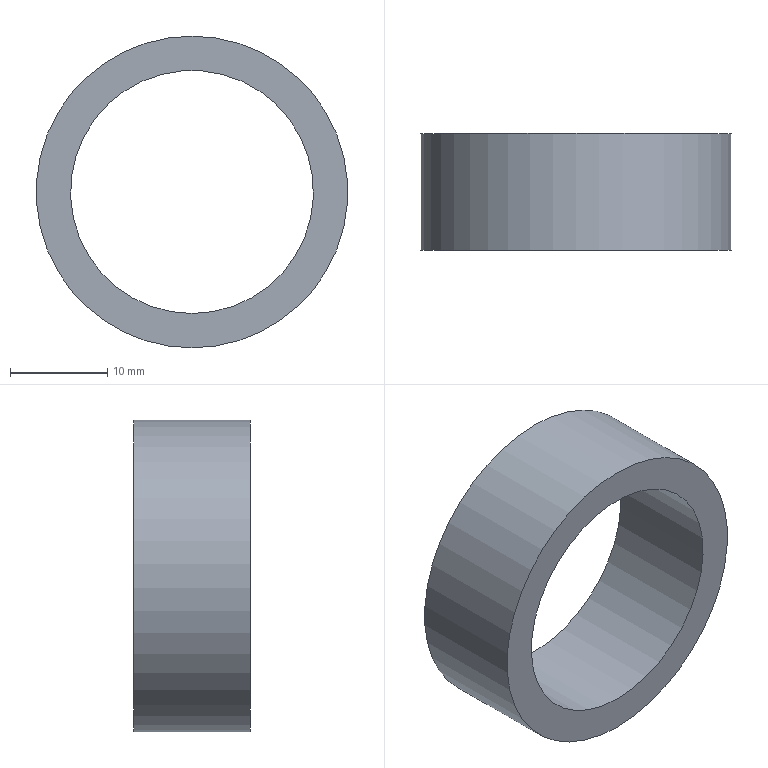Component | NX | SLEEVE | 1 solid | 4 faces | box 32.07 x 12 x 32.07 mm | volume 3803 mm3 | cylinder 2 | plane 2 | commonest cylinder face diameters 32.07 x1 25 x1
STEP:
#1=CARTESIAN_POINT('',(0.,0.,0.));
#2=DIRECTION('',(0.,0.,1.));
#3=DIRECTION('',(1.,0.,0.));
#4=AXIS2_PLACEMENT_3D('',#1,#2,#3);
#5=CARTESIAN_POINT('',(0.,-34.96,-16.035));
#6=VERTEX_POINT('',#5);
#7=CARTESIAN_POINT('',(0.,-34.96,0.));
#8=DIRECTION('',(0.,-1.,0.));
#9=DIRECTION('',(0.,0.,-1.));
#10=AXIS2_PLACEMENT_3D('',#7,#8,#9);
#11=CIRCLE('',#10,16.035);
#12=CARTESIAN_POINT('',(0.,0.,0.));
#13=DIRECTION('',(0.,-1.,0.));
#14=DIRECTION('',(0.,0.,-1.));
#15=AXIS2_PLACEMENT_3D('',#12,#13,#14);
#16=CYLINDRICAL_SURFACE('',#15,16.035);
#17=CARTESIAN_POINT('',(0.,34.96));
#18=DIRECTION('',(1.,0.));
#19=VECTOR('',#18,1.);
#20=LINE('',#17,#19);
#21=(GEOMETRIC_REPRESENTATION_CONTEXT(2)PARAMETRIC_REPRESENTATION_CONTEXT()REPRESENTATION_CONTEXT('',''));
#22=DEFINITIONAL_REPRESENTATION('',(#20),#21);
#23=PCURVE('',#16,#22);
#24=CARTESIAN_POINT('',(-16.035,-34.96,0.));
#25=DIRECTION('',(0.,1.,0.));
#26=DIRECTION('',(0.,0.,1.));
#27=AXIS2_PLACEMENT_3D('',#24,#25,#26);
#28=PLANE('',#27);
#29=CARTESIAN_POINT('',(-16.035,16.035));
#30=CARTESIAN_POINT('',(-16.035,43.808));
#31=CARTESIAN_POINT('',(8.017,29.922));
#32=CARTESIAN_POINT('',(32.07,16.035));
#33=CARTESIAN_POINT('',(8.017,2.148));
#34=CARTESIAN_POINT('',(-16.035,-11.738));
#35=CARTESIAN_POINT('',(-16.035,16.035));
#36=(BOUNDED_CURVE()B_SPLINE_CURVE(2,(#29,#30,#31,#32,#33,#34,#35),.UNSPECIFIED.,.T.,.F.)B_SPLINE_CURVE_WITH_KNOTS((1,2,2,2,2,1),(-2.094,0.,2.094,4.189,6.283,8.378),.UNSPECIFIED.)CURVE()GEOMETRIC_REPRESENTATION_ITEM()RATIONAL_B_SPLINE_CURVE((1.,0.5,1.,0.5,1.,0.5,1.))REPRESENTATION_ITEM(''));
#37=(GEOMETRIC_REPRESENTATION_CONTEXT(2)PARAMETRIC_REPRESENTATION_CONTEXT()REPRESENTATION_CONTEXT('',''));
#38=DEFINITIONAL_REPRESENTATION('',(#36),#37);
#39=PCURVE('',#28,#38);
#40=SURFACE_CURVE('',#11,(#23,#39),.PCURVE_S1.);
#41=EDGE_CURVE('',#6,#6,#40,.T.);
#42=ORIENTED_EDGE('',*,*,#41,.F.);
#43=CARTESIAN_POINT('',(0.,-22.96,-16.035));
#44=VERTEX_POINT('',#43);
#45=CARTESIAN_POINT('',(-0.,-22.96,-16.035));
#46=CARTESIAN_POINT('',(-0.,-34.96,-16.035));
#47=B_SPLINE_CURVE_WITH_KNOTS('',1,(#45,#46),.UNSPECIFIED.,.F.,.F.,(2,2),(22.96,34.96),.PIECEWISE_BEZIER_KNOTS.);
#48=CARTESIAN_POINT('',(0.,0.));
#49=DIRECTION('',(0.,1.));
#50=VECTOR('',#49,1.);
#51=LINE('',#48,#50);
#52=(GEOMETRIC_REPRESENTATION_CONTEXT(2)PARAMETRIC_REPRESENTATION_CONTEXT()REPRESENTATION_CONTEXT('',''));
#53=DEFINITIONAL_REPRESENTATION('',(#51),#52);
#54=PCURVE('',#16,#53);
#55=CARTESIAN_POINT('',(6.283,0.));
#56=DIRECTION('',(0.,1.));
#57=VECTOR('',#56,1.);
#58=LINE('',#55,#57);
#59=(GEOMETRIC_REPRESENTATION_CONTEXT(2)PARAMETRIC_REPRESENTATION_CONTEXT()REPRESENTATION_CONTEXT('',''));
#60=DEFINITIONAL_REPRESENTATION('',(#58),#59);
#61=PCURVE('',#16,#60);
#62=SEAM_CURVE('',#47,(#54,#61),.PCURVE_S1.);
#63=EDGE_CURVE('',#44,#6,#62,.T.);
#64=ORIENTED_EDGE('',*,*,#63,.F.);
#65=CARTESIAN_POINT('',(0.,-22.96,0.));
#66=DIRECTION('',(0.,-1.,0.));
#67=DIRECTION('',(0.,0.,-1.));
#68=AXIS2_PLACEMENT_3D('',#65,#66,#67);
#69=CIRCLE('',#68,16.035);
#70=CARTESIAN_POINT('',(0.,22.96));
#71=DIRECTION('',(1.,0.));
#72=VECTOR('',#71,1.);
#73=LINE('',#70,#72);
#74=(GEOMETRIC_REPRESENTATION_CONTEXT(2)PARAMETRIC_REPRESENTATION_CONTEXT()REPRESENTATION_CONTEXT('',''));
#75=DEFINITIONAL_REPRESENTATION('',(#73),#74);
#76=PCURVE('',#16,#75);
#77=CARTESIAN_POINT('',(-12.5,-22.96,0.));
#78=DIRECTION('',(0.,-1.,0.));
#79=DIRECTION('',(0.,0.,-1.));
#80=AXIS2_PLACEMENT_3D('',#77,#78,#79);
#81=PLANE('',#80);
#82=CARTESIAN_POINT('',(0.,12.5));
#83=DIRECTION('',(1.,0.));
#84=AXIS2_PLACEMENT_2D('',#82,#83);
#85=CIRCLE('',#84,16.035);
#86=(GEOMETRIC_REPRESENTATION_CONTEXT(2)PARAMETRIC_REPRESENTATION_CONTEXT()REPRESENTATION_CONTEXT('',''));
#87=DEFINITIONAL_REPRESENTATION('',(#85),#86);
#88=PCURVE('',#81,#87);
#89=SURFACE_CURVE('',#69,(#76,#88),.PCURVE_S1.);
#90=EDGE_CURVE('',#44,#44,#89,.T.);
#91=ORIENTED_EDGE('',*,*,#90,.T.);
#92=ORIENTED_EDGE('',*,*,#63,.T.);
#93=EDGE_LOOP('',(#42,#64,#91,#92));
#94=FACE_BOUND('',#93,.T.);
#95=ADVANCED_FACE('',(#94),#16,.T.);
#96=CARTESIAN_POINT('',(0.,-34.96,-12.5));
#97=VERTEX_POINT('',#96);
#98=CARTESIAN_POINT('',(0.,-34.96,0.));
#99=DIRECTION('',(0.,-1.,0.));
#100=DIRECTION('',(0.,0.,-1.));
#101=AXIS2_PLACEMENT_3D('',#98,#99,#100);
#102=CIRCLE('',#101,12.5);
#103=CARTESIAN_POINT('',(-12.5,16.035));
#104=CARTESIAN_POINT('',(-12.5,37.686));
#105=CARTESIAN_POINT('',(6.25,26.86));
#106=CARTESIAN_POINT('',(25.,16.035));
#107=CARTESIAN_POINT('',(6.25,5.21));
#108=CARTESIAN_POINT('',(-12.5,-5.616));
#109=CARTESIAN_POINT('',(-12.5,16.035));
#110=(BOUNDED_CURVE()B_SPLINE_CURVE(2,(#103,#104,#105,#106,#107,#108,#109),.UNSPECIFIED.,.T.,.F.)B_SPLINE_CURVE_WITH_KNOTS((1,2,2,2,2,1),(-2.094,0.,2.094,4.189,6.283,8.378),.UNSPECIFIED.)CURVE()GEOMETRIC_REPRESENTATION_ITEM()RATIONAL_B_SPLINE_CURVE((1.,0.5,1.,0.5,1.,0.5,1.))REPRESENTATION_ITEM(''));
#111=(GEOMETRIC_REPRESENTATION_CONTEXT(2)PARAMETRIC_REPRESENTATION_CONTEXT()REPRESENTATION_CONTEXT('',''));
#112=DEFINITIONAL_REPRESENTATION('',(#110),#111);
#113=PCURVE('',#28,#112);
#114=CARTESIAN_POINT('',(0.,0.,0.));
#115=DIRECTION('',(0.,-1.,0.));
#116=DIRECTION('',(0.,0.,-1.));
#117=AXIS2_PLACEMENT_3D('',#114,#115,#116);
#118=CYLINDRICAL_SURFACE('',#117,12.5);
#119=CARTESIAN_POINT('',(0.,34.96));
#120=DIRECTION('',(1.,0.));
#121=VECTOR('',#120,1.);
#122=LINE('',#119,#121);
#123=(GEOMETRIC_REPRESENTATION_CONTEXT(2)PARAMETRIC_REPRESENTATION_CONTEXT()REPRESENTATION_CONTEXT('',''));
#124=DEFINITIONAL_REPRESENTATION('',(#122),#123);
#125=PCURVE('',#118,#124);
#126=SURFACE_CURVE('',#102,(#113,#125),.PCURVE_S1.);
#127=EDGE_CURVE('',#97,#97,#126,.T.);
#128=ORIENTED_EDGE('',*,*,#127,.F.);
#129=EDGE_LOOP('',(#128));
#130=FACE_BOUND('',#129,.T.);
#131=ORIENTED_EDGE('',*,*,#41,.T.);
#132=EDGE_LOOP('',(#131));
#133=FACE_BOUND('',#132,.T.);
#134=ADVANCED_FACE('',(#130,#133),#28,.F.);
#135=CARTESIAN_POINT('',(0.,-22.96,-12.5));
#136=VERTEX_POINT('',#135);
#137=CARTESIAN_POINT('',(0.,-22.96,0.));
#138=DIRECTION('',(0.,-1.,0.));
#139=DIRECTION('',(0.,0.,-1.));
#140=AXIS2_PLACEMENT_3D('',#137,#138,#139);
#141=CIRCLE('',#140,12.5);
#142=CARTESIAN_POINT('',(0.,22.96));
#143=DIRECTION('',(1.,0.));
#144=VECTOR('',#143,1.);
#145=LINE('',#142,#144);
#146=(GEOMETRIC_REPRESENTATION_CONTEXT(2)PARAMETRIC_REPRESENTATION_CONTEXT()REPRESENTATION_CONTEXT('',''));
#147=DEFINITIONAL_REPRESENTATION('',(#145),#146);
#148=PCURVE('',#118,#147);
#149=CARTESIAN_POINT('',(0.,12.5));
#150=DIRECTION('',(1.,0.));
#151=AXIS2_PLACEMENT_2D('',#149,#150);
#152=CIRCLE('',#151,12.5);
#153=(GEOMETRIC_REPRESENTATION_CONTEXT(2)PARAMETRIC_REPRESENTATION_CONTEXT()REPRESENTATION_CONTEXT('',''));
#154=DEFINITIONAL_REPRESENTATION('',(#152),#153);
#155=PCURVE('',#81,#154);
#156=SURFACE_CURVE('',#141,(#148,#155),.PCURVE_S1.);
#157=EDGE_CURVE('',#136,#136,#156,.T.);
#158=ORIENTED_EDGE('',*,*,#157,.T.);
#159=CARTESIAN_POINT('',(0.,-22.96,-12.5));
#160=CARTESIAN_POINT('',(0.,-34.96,-12.5));
#161=B_SPLINE_CURVE_WITH_KNOTS('',1,(#159,#160),.UNSPECIFIED.,.F.,.F.,(2,2),(22.96,34.96),.PIECEWISE_BEZIER_KNOTS.);
#162=CARTESIAN_POINT('',(6.283,0.));
#163=DIRECTION('',(0.,1.));
#164=VECTOR('',#163,1.);
#165=LINE('',#162,#164);
#166=(GEOMETRIC_REPRESENTATION_CONTEXT(2)PARAMETRIC_REPRESENTATION_CONTEXT()REPRESENTATION_CONTEXT('',''));
#167=DEFINITIONAL_REPRESENTATION('',(#165),#166);
#168=PCURVE('',#118,#167);
#169=CARTESIAN_POINT('',(0.,0.));
#170=DIRECTION('',(0.,1.));
#171=VECTOR('',#170,1.);
#172=LINE('',#169,#171);
#173=(GEOMETRIC_REPRESENTATION_CONTEXT(2)PARAMETRIC_REPRESENTATION_CONTEXT()REPRESENTATION_CONTEXT('',''));
#174=DEFINITIONAL_REPRESENTATION('',(#172),#173);
#175=PCURVE('',#118,#174);
#176=SEAM_CURVE('',#161,(#168,#175),.PCURVE_S1.);
#177=EDGE_CURVE('',#136,#97,#176,.T.);
#178=ORIENTED_EDGE('',*,*,#177,.T.);
#179=ORIENTED_EDGE('',*,*,#127,.F.);
#180=ORIENTED_EDGE('',*,*,#177,.F.);
#181=EDGE_LOOP('',(#158,#178,#179,#180));
#182=FACE_BOUND('',#181,.F.);
#183=ADVANCED_FACE('',(#182),#118,.F.);
#184=ORIENTED_EDGE('',*,*,#90,.F.);
#185=EDGE_LOOP('',(#184));
#186=FACE_BOUND('',#185,.T.);
#187=ORIENTED_EDGE('',*,*,#157,.T.);
#188=EDGE_LOOP('',(#187));
#189=FACE_BOUND('',#188,.T.);
#190=ADVANCED_FACE('',(#186,#189),#81,.F.);
#191=CLOSED_SHELL('',(#95,#134,#183,#190));
#192=MANIFOLD_SOLID_BREP('',#191);
#193=(LENGTH_UNIT()NAMED_UNIT(*)SI_UNIT(.MILLI.,.METRE.));
#194=UNCERTAINTY_MEASURE_WITH_UNIT(LENGTH_MEASURE(0.00001),#193,'','');
#195=(NAMED_UNIT(*)PLANE_ANGLE_UNIT()SI_UNIT($,.RADIAN.));
#196=(NAMED_UNIT(*)SI_UNIT($,.STERADIAN.)SOLID_ANGLE_UNIT());
#197=(GEOMETRIC_REPRESENTATION_CONTEXT(3)GLOBAL_UNCERTAINTY_ASSIGNED_CONTEXT((#194))GLOBAL_UNIT_ASSIGNED_CONTEXT((#193,#195,#196))REPRESENTATION_CONTEXT('',''));
#198=ADVANCED_BREP_SHAPE_REPRESENTATION('',(#4,#192),#197);